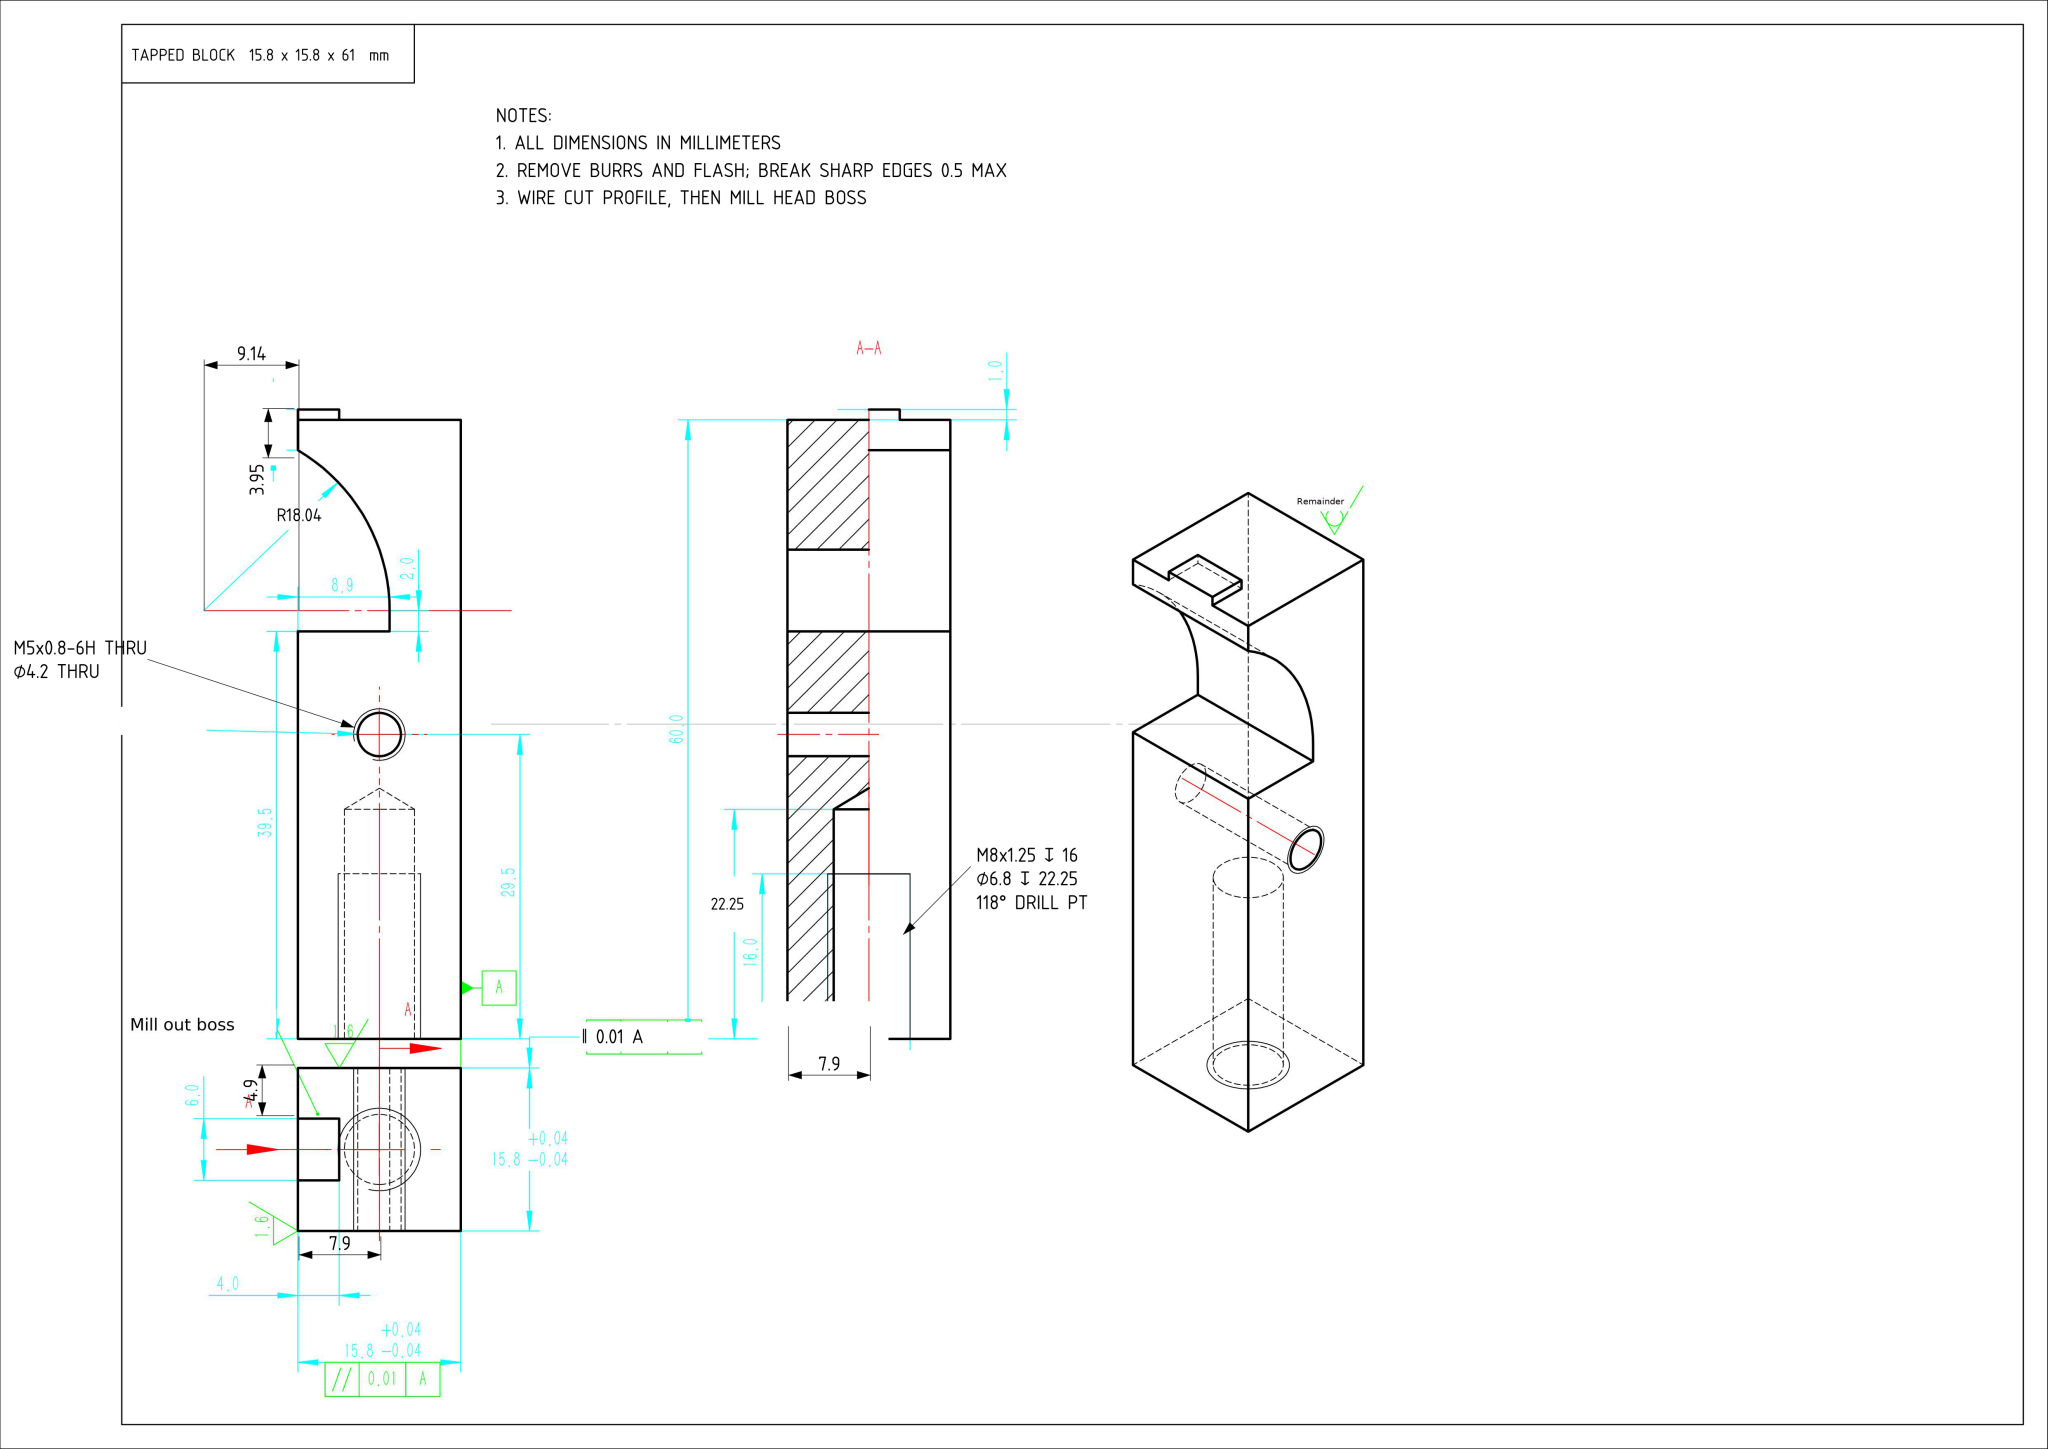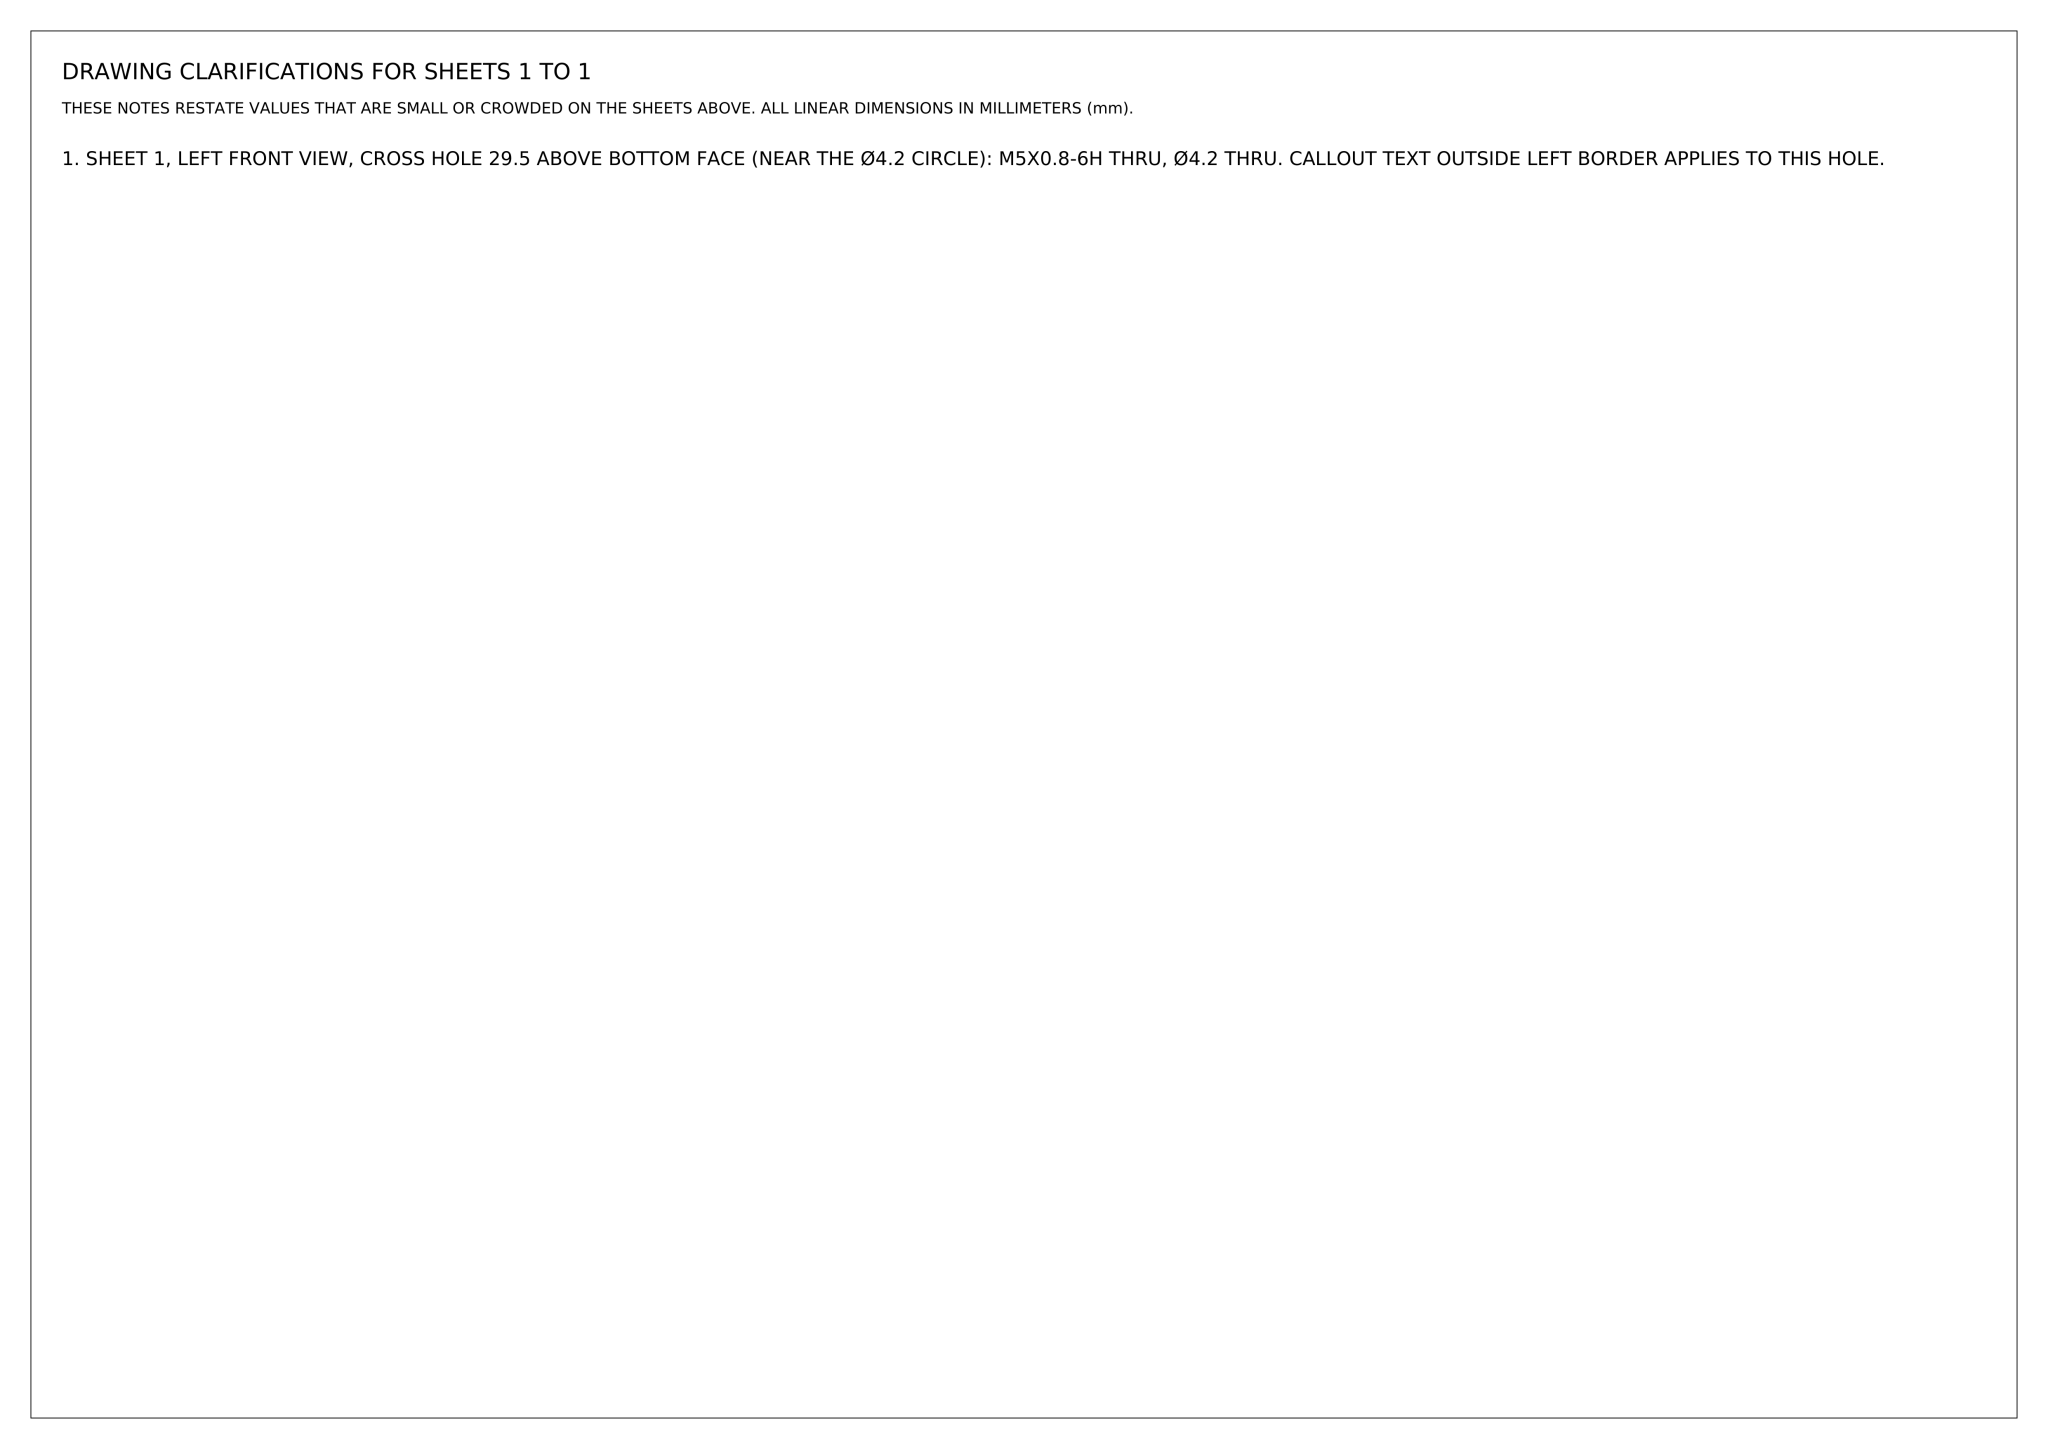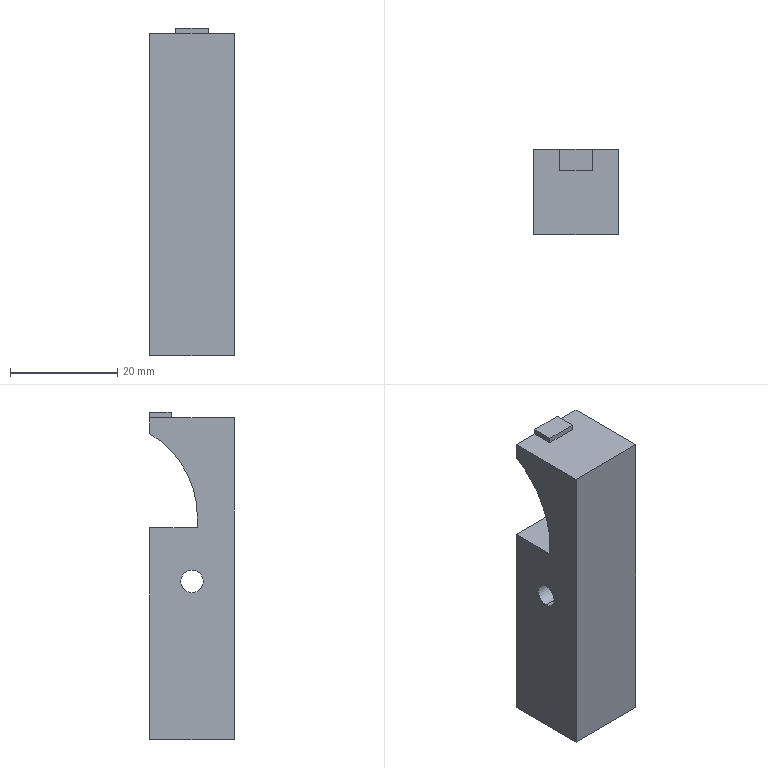Part | NX | mm | 1 solid | 20 faces | box 15.8 x 15.8 x 61 mm | volume 12120 mm3 | plane 13 | cylinder 5 | cone 2 | commonest cylinder face diameters 4.2 x2 6.8 x2 36.083 x1
STEP:
#1=COLOUR_RGB('',1.,0.651,0.);
#2=FILL_AREA_STYLE_COLOUR('',#1);
#3=FILL_AREA_STYLE('',(#2));
#4=SURFACE_STYLE_FILL_AREA(#3);
#5=SURFACE_SIDE_STYLE('',(#4));
#6=SURFACE_STYLE_USAGE(.BOTH.,#5);
#7=PRESENTATION_STYLE_ASSIGNMENT((#6));
#8=CARTESIAN_POINT('',(0.01211,-22.1,27.4));
#9=VERTEX_POINT('',#8);
#10=CARTESIAN_POINT('',(0.01211,-22.1,31.6));
#11=VERTEX_POINT('',#10);
#12=CARTESIAN_POINT('',(0.01211,-22.1,29.5));
#13=DIRECTION('',(-1.,-0.,0.));
#14=DIRECTION('',(0.,-1.,0.));
#15=AXIS2_PLACEMENT_3D('',#12,#13,#14);
#16=CIRCLE('',#15,2.1);
#17=EDGE_CURVE('',#9,#11,#16,.T.);
#18=ORIENTED_EDGE('',*,*,#17,.F.);
#19=CARTESIAN_POINT('',(-15.788,-22.1,27.4));
#20=VERTEX_POINT('',#19);
#21=CARTESIAN_POINT('',(-15.788,-22.1,27.4));
#22=DIRECTION('',(-1.,0.,0.));
#23=VECTOR('',#22,1000.);
#24=LINE('',#21,#23);
#25=EDGE_CURVE('',#9,#20,#24,.T.);
#26=ORIENTED_EDGE('',*,*,#25,.T.);
#27=CARTESIAN_POINT('',(-15.788,-22.1,31.6));
#28=VERTEX_POINT('',#27);
#29=CARTESIAN_POINT('',(-15.788,-22.1,29.5));
#30=DIRECTION('',(-1.,0.,0.));
#31=DIRECTION('',(0.,0.,1.));
#32=AXIS2_PLACEMENT_3D('',#29,#30,#31);
#33=CIRCLE('',#32,2.1);
#34=EDGE_CURVE('',#20,#28,#33,.T.);
#35=ORIENTED_EDGE('',*,*,#34,.T.);
#36=CARTESIAN_POINT('',(-15.788,-22.1,31.6));
#37=DIRECTION('',(-1.,0.,0.));
#38=VECTOR('',#37,1000.);
#39=LINE('',#36,#38);
#40=EDGE_CURVE('',#11,#28,#39,.T.);
#41=ORIENTED_EDGE('',*,*,#40,.F.);
#42=EDGE_LOOP('',(#18,#26,#35,#41));
#43=FACE_OUTER_BOUND('',#42,.T.);
#44=CARTESIAN_POINT('',(-15.788,-22.1,29.5));
#45=DIRECTION('',(-1.,0.,0.));
#46=DIRECTION('',(0.,0.,1.));
#47=AXIS2_PLACEMENT_3D('',#44,#45,#46);
#48=CYLINDRICAL_SURFACE('',#47,2.1);
#49=ADVANCED_FACE('',(#43),#48,.F.);
#50=CARTESIAN_POINT('',(-4.488,-22.1,22.25));
#51=VERTEX_POINT('',#50);
#52=CARTESIAN_POINT('',(-11.288,-22.1,22.25));
#53=VERTEX_POINT('',#52);
#54=CARTESIAN_POINT('',(-7.888,-22.1,22.25));
#55=DIRECTION('',(0.,0.,-1.));
#56=DIRECTION('',(-1.,0.,0.));
#57=AXIS2_PLACEMENT_3D('',#54,#55,#56);
#58=CIRCLE('',#57,3.4);
#59=EDGE_CURVE('',#51,#53,#58,.T.);
#60=ORIENTED_EDGE('',*,*,#59,.F.);
#61=CARTESIAN_POINT('',(-4.488,-22.1,-0.));
#62=VERTEX_POINT('',#61);
#63=CARTESIAN_POINT('',(-4.488,-22.1,0.));
#64=DIRECTION('',(0.,0.,-1.));
#65=VECTOR('',#64,1000.);
#66=LINE('',#63,#65);
#67=EDGE_CURVE('',#51,#62,#66,.T.);
#68=ORIENTED_EDGE('',*,*,#67,.T.);
#69=CARTESIAN_POINT('',(-11.288,-22.1,-0.));
#70=VERTEX_POINT('',#69);
#71=CARTESIAN_POINT('',(-7.888,-22.1,-0.));
#72=DIRECTION('',(0.,0.,-1.));
#73=DIRECTION('',(-1.,0.,0.));
#74=AXIS2_PLACEMENT_3D('',#71,#72,#73);
#75=CIRCLE('',#74,3.4);
#76=EDGE_CURVE('',#62,#70,#75,.T.);
#77=ORIENTED_EDGE('',*,*,#76,.T.);
#78=CARTESIAN_POINT('',(-11.288,-22.1,0.));
#79=DIRECTION('',(0.,0.,-1.));
#80=VECTOR('',#79,1000.);
#81=LINE('',#78,#80);
#82=EDGE_CURVE('',#53,#70,#81,.T.);
#83=ORIENTED_EDGE('',*,*,#82,.F.);
#84=EDGE_LOOP('',(#60,#68,#77,#83));
#85=FACE_OUTER_BOUND('',#84,.T.);
#86=CARTESIAN_POINT('',(-7.888,-22.1,0.));
#87=DIRECTION('',(0.,0.,-1.));
#88=DIRECTION('',(-1.,0.,0.));
#89=AXIS2_PLACEMENT_3D('',#86,#87,#88);
#90=CYLINDRICAL_SURFACE('',#89,3.4);
#91=ADVANCED_FACE('',(#85),#90,.F.);
#92=CARTESIAN_POINT('',(-7.888,-22.1,24.293));
#93=VERTEX_POINT('',#92);
#94=CARTESIAN_POINT('',(-11.288,-22.1,22.25));
#95=DIRECTION('',(-0.8572,0.,-0.515));
#96=VECTOR('',#95,1000.);
#97=LINE('',#94,#96);
#98=EDGE_CURVE('',#93,#53,#97,.T.);
#99=ORIENTED_EDGE('',*,*,#98,.F.);
#100=CARTESIAN_POINT('',(-4.488,-22.1,22.25));
#101=DIRECTION('',(0.8572,0.,-0.515));
#102=VECTOR('',#101,1000.);
#103=LINE('',#100,#102);
#104=EDGE_CURVE('',#93,#51,#103,.T.);
#105=ORIENTED_EDGE('',*,*,#104,.T.);
#106=ORIENTED_EDGE('',*,*,#59,.T.);
#107=EDGE_LOOP('',(#99,#105,#106));
#108=FACE_OUTER_BOUND('',#107,.T.);
#109=CARTESIAN_POINT('',(-7.888,-22.1,22.25));
#110=DIRECTION('',(0.,0.,-1.));
#111=DIRECTION('',(-1.,0.,0.));
#112=AXIS2_PLACEMENT_3D('',#109,#110,#111);
#113=CONICAL_SURFACE('',#112,3.4,1.03);
#114=ADVANCED_FACE('',(#108),#113,.F.);
#115=CARTESIAN_POINT('',(-10.888,-14.2,60.));
#116=VERTEX_POINT('',#115);
#117=CARTESIAN_POINT('',(-10.888,-18.2,60.));
#118=VERTEX_POINT('',#117);
#119=CARTESIAN_POINT('',(-10.888,-14.2,60.));
#120=DIRECTION('',(0.,-1.,0.));
#121=VECTOR('',#120,1000.);
#122=LINE('',#119,#121);
#123=EDGE_CURVE('',#116,#118,#122,.T.);
#124=ORIENTED_EDGE('',*,*,#123,.F.);
#125=CARTESIAN_POINT('',(-15.788,-14.2,60.));
#126=VERTEX_POINT('',#125);
#127=CARTESIAN_POINT('',(0.01211,-14.2,60.));
#128=DIRECTION('',(-1.,-0.,0.));
#129=VECTOR('',#128,1000.);
#130=LINE('',#127,#129);
#131=EDGE_CURVE('',#116,#126,#130,.T.);
#132=ORIENTED_EDGE('',*,*,#131,.T.);
#133=CARTESIAN_POINT('',(-15.788,-30.,60.));
#134=VERTEX_POINT('',#133);
#135=CARTESIAN_POINT('',(-15.788,-14.2,60.));
#136=DIRECTION('',(0.,-1.,0.));
#137=VECTOR('',#136,1000.);
#138=LINE('',#135,#137);
#139=EDGE_CURVE('',#126,#134,#138,.T.);
#140=ORIENTED_EDGE('',*,*,#139,.T.);
#141=CARTESIAN_POINT('',(0.01211,-30.,60.));
#142=VERTEX_POINT('',#141);
#143=CARTESIAN_POINT('',(0.01211,-30.,60.));
#144=DIRECTION('',(1.,0.,0.));
#145=VECTOR('',#144,1000.);
#146=LINE('',#143,#145);
#147=EDGE_CURVE('',#134,#142,#146,.T.);
#148=ORIENTED_EDGE('',*,*,#147,.T.);
#149=CARTESIAN_POINT('',(0.01211,-14.2,60.));
#150=VERTEX_POINT('',#149);
#151=CARTESIAN_POINT('',(0.01211,-14.2,60.));
#152=DIRECTION('',(-0.,1.,0.));
#153=VECTOR('',#152,1000.);
#154=LINE('',#151,#153);
#155=EDGE_CURVE('',#142,#150,#154,.T.);
#156=ORIENTED_EDGE('',*,*,#155,.T.);
#157=CARTESIAN_POINT('',(-4.888,-14.2,60.));
#158=VERTEX_POINT('',#157);
#159=CARTESIAN_POINT('',(0.01211,-14.2,60.));
#160=DIRECTION('',(-1.,-0.,0.));
#161=VECTOR('',#160,1000.);
#162=LINE('',#159,#161);
#163=EDGE_CURVE('',#150,#158,#162,.T.);
#164=ORIENTED_EDGE('',*,*,#163,.T.);
#165=CARTESIAN_POINT('',(-4.888,-18.2,60.));
#166=VERTEX_POINT('',#165);
#167=CARTESIAN_POINT('',(-4.888,-14.2,60.));
#168=DIRECTION('',(0.,-1.,0.));
#169=VECTOR('',#168,1000.);
#170=LINE('',#167,#169);
#171=EDGE_CURVE('',#158,#166,#170,.T.);
#172=ORIENTED_EDGE('',*,*,#171,.T.);
#173=CARTESIAN_POINT('',(-10.888,-18.2,60.));
#174=DIRECTION('',(1.,0.,0.));
#175=VECTOR('',#174,1000.);
#176=LINE('',#173,#175);
#177=EDGE_CURVE('',#118,#166,#176,.T.);
#178=ORIENTED_EDGE('',*,*,#177,.F.);
#179=EDGE_LOOP('',(#124,#132,#140,#148,#156,#164,#172,#178));
#180=FACE_OUTER_BOUND('',#179,.T.);
#181=CARTESIAN_POINT('',(0.,0.,60.));
#182=DIRECTION('',(0.,0.,-1.));
#183=DIRECTION('',(-1.,0.,0.));
#184=AXIS2_PLACEMENT_3D('',#181,#182,#183);
#185=PLANE('',#184);
#186=ADVANCED_FACE('',(#180),#185,.F.);
#187=CARTESIAN_POINT('',(-15.788,-23.1,41.5));
#188=VERTEX_POINT('',#187);
#189=CARTESIAN_POINT('',(-15.788,-14.2,57.054));
#190=VERTEX_POINT('',#189);
#191=CARTESIAN_POINT('',(-15.788,-5.058,41.5));
#192=DIRECTION('',(-1.,0.,0.));
#193=DIRECTION('',(0.,0.,1.));
#194=AXIS2_PLACEMENT_3D('',#191,#192,#193);
#195=CIRCLE('',#194,18.042);
#196=EDGE_CURVE('',#188,#190,#195,.T.);
#197=ORIENTED_EDGE('',*,*,#196,.F.);
#198=CARTESIAN_POINT('',(-15.788,-23.1,39.5));
#199=VERTEX_POINT('',#198);
#200=CARTESIAN_POINT('',(-15.788,-23.1,41.5));
#201=DIRECTION('',(0.,0.,1.));
#202=VECTOR('',#201,1000.);
#203=LINE('',#200,#202);
#204=EDGE_CURVE('',#199,#188,#203,.T.);
#205=ORIENTED_EDGE('',*,*,#204,.F.);
#206=CARTESIAN_POINT('',(-15.788,-14.2,39.5));
#207=VERTEX_POINT('',#206);
#208=CARTESIAN_POINT('',(-15.788,-14.2,39.5));
#209=DIRECTION('',(0.,-1.,0.));
#210=VECTOR('',#209,1000.);
#211=LINE('',#208,#210);
#212=EDGE_CURVE('',#207,#199,#211,.T.);
#213=ORIENTED_EDGE('',*,*,#212,.F.);
#214=CARTESIAN_POINT('',(-15.788,-14.2,0.));
#215=VERTEX_POINT('',#214);
#216=CARTESIAN_POINT('',(-15.788,-14.2,60.));
#217=DIRECTION('',(0.,0.,-1.));
#218=VECTOR('',#217,1000.);
#219=LINE('',#216,#218);
#220=EDGE_CURVE('',#207,#215,#219,.T.);
#221=ORIENTED_EDGE('',*,*,#220,.T.);
#222=CARTESIAN_POINT('',(-15.788,-30.,0.));
#223=VERTEX_POINT('',#222);
#224=CARTESIAN_POINT('',(-15.788,-14.2,0.));
#225=DIRECTION('',(0.,-1.,0.));
#226=VECTOR('',#225,1000.);
#227=LINE('',#224,#226);
#228=EDGE_CURVE('',#215,#223,#227,.T.);
#229=ORIENTED_EDGE('',*,*,#228,.T.);
#230=CARTESIAN_POINT('',(-15.788,-30.,60.));
#231=DIRECTION('',(0.,0.,-1.));
#232=VECTOR('',#231,1000.);
#233=LINE('',#230,#232);
#234=EDGE_CURVE('',#134,#223,#233,.T.);
#235=ORIENTED_EDGE('',*,*,#234,.F.);
#236=ORIENTED_EDGE('',*,*,#139,.F.);
#237=CARTESIAN_POINT('',(-15.788,-14.2,60.));
#238=DIRECTION('',(0.,0.,-1.));
#239=VECTOR('',#238,1000.);
#240=LINE('',#237,#239);
#241=EDGE_CURVE('',#126,#190,#240,.T.);
#242=ORIENTED_EDGE('',*,*,#241,.T.);
#243=EDGE_LOOP('',(#197,#205,#213,#221,#229,#235,#236,#242));
#244=FACE_OUTER_BOUND('',#243,.T.);
#245=CARTESIAN_POINT('',(-15.788,-22.1,29.5));
#246=DIRECTION('',(-1.,0.,0.));
#247=DIRECTION('',(0.,0.,1.));
#248=AXIS2_PLACEMENT_3D('',#245,#246,#247);
#249=CIRCLE('',#248,2.1);
#250=EDGE_CURVE('',#28,#20,#249,.T.);
#251=ORIENTED_EDGE('',*,*,#250,.F.);
#252=ORIENTED_EDGE('',*,*,#34,.F.);
#253=EDGE_LOOP('',(#251,#252));
#254=FACE_BOUND('',#253,.T.);
#255=CARTESIAN_POINT('',(-15.788,-14.2,60.));
#256=DIRECTION('',(1.,0.,0.));
#257=DIRECTION('',(0.,0.,-1.));
#258=AXIS2_PLACEMENT_3D('',#255,#256,#257);
#259=PLANE('',#258);
#260=ADVANCED_FACE('',(#244,#254),#259,.F.);
#261=CARTESIAN_POINT('',(0.01211,-14.2,57.054));
#262=VERTEX_POINT('',#261);
#263=CARTESIAN_POINT('',(0.01211,-14.2,60.));
#264=DIRECTION('',(0.,0.,-1.));
#265=VECTOR('',#264,1000.);
#266=LINE('',#263,#265);
#267=EDGE_CURVE('',#150,#262,#266,.T.);
#268=ORIENTED_EDGE('',*,*,#267,.T.);
#269=CARTESIAN_POINT('',(0.01311,-14.2,57.054));
#270=DIRECTION('',(1.,0.,0.));
#271=VECTOR('',#270,1000.);
#272=LINE('',#269,#271);
#273=EDGE_CURVE('',#190,#262,#272,.T.);
#274=ORIENTED_EDGE('',*,*,#273,.F.);
#275=ORIENTED_EDGE('',*,*,#241,.F.);
#276=ORIENTED_EDGE('',*,*,#131,.F.);
#277=CARTESIAN_POINT('',(-10.888,-14.2,61.));
#278=VERTEX_POINT('',#277);
#279=CARTESIAN_POINT('',(-10.888,-14.2,61.));
#280=DIRECTION('',(0.,0.,-1.));
#281=VECTOR('',#280,1000.);
#282=LINE('',#279,#281);
#283=EDGE_CURVE('',#278,#116,#282,.T.);
#284=ORIENTED_EDGE('',*,*,#283,.F.);
#285=CARTESIAN_POINT('',(-4.888,-14.2,61.));
#286=VERTEX_POINT('',#285);
#287=CARTESIAN_POINT('',(-10.888,-14.2,61.));
#288=DIRECTION('',(1.,0.,0.));
#289=VECTOR('',#288,1000.);
#290=LINE('',#287,#289);
#291=EDGE_CURVE('',#278,#286,#290,.T.);
#292=ORIENTED_EDGE('',*,*,#291,.T.);
#293=CARTESIAN_POINT('',(-4.888,-14.2,61.));
#294=DIRECTION('',(0.,0.,-1.));
#295=VECTOR('',#294,1000.);
#296=LINE('',#293,#295);
#297=EDGE_CURVE('',#286,#158,#296,.T.);
#298=ORIENTED_EDGE('',*,*,#297,.T.);
#299=ORIENTED_EDGE('',*,*,#163,.F.);
#300=EDGE_LOOP('',(#268,#274,#275,#276,#284,#292,#298,#299));
#301=FACE_OUTER_BOUND('',#300,.T.);
#302=CARTESIAN_POINT('',(0.01211,-14.2,60.));
#303=DIRECTION('',(0.,-1.,0.));
#304=DIRECTION('',(1.,0.,0.));
#305=AXIS2_PLACEMENT_3D('',#302,#303,#304);
#306=PLANE('',#305);
#307=ADVANCED_FACE('',(#301),#306,.F.);
#308=CARTESIAN_POINT('',(0.01211,-22.1,29.5));
#309=DIRECTION('',(-1.,-0.,0.));
#310=DIRECTION('',(0.,-1.,0.));
#311=AXIS2_PLACEMENT_3D('',#308,#309,#310);
#312=CIRCLE('',#311,2.1);
#313=EDGE_CURVE('',#11,#9,#312,.T.);
#314=ORIENTED_EDGE('',*,*,#313,.T.);
#315=ORIENTED_EDGE('',*,*,#17,.T.);
#316=EDGE_LOOP('',(#314,#315));
#317=FACE_BOUND('',#316,.T.);
#318=CARTESIAN_POINT('',(0.01211,-14.2,39.5));
#319=VERTEX_POINT('',#318);
#320=CARTESIAN_POINT('',(0.01211,-23.1,39.5));
#321=VERTEX_POINT('',#320);
#322=CARTESIAN_POINT('',(0.01211,-14.2,39.5));
#323=DIRECTION('',(0.,-1.,0.));
#324=VECTOR('',#323,1000.);
#325=LINE('',#322,#324);
#326=EDGE_CURVE('',#319,#321,#325,.T.);
#327=ORIENTED_EDGE('',*,*,#326,.T.);
#328=CARTESIAN_POINT('',(0.01211,-23.1,41.5));
#329=VERTEX_POINT('',#328);
#330=CARTESIAN_POINT('',(0.01211,-23.1,60.));
#331=DIRECTION('',(0.,0.,1.));
#332=VECTOR('',#331,1000.);
#333=LINE('',#330,#332);
#334=EDGE_CURVE('',#321,#329,#333,.T.);
#335=ORIENTED_EDGE('',*,*,#334,.T.);
#336=CARTESIAN_POINT('',(0.01211,-5.058,41.5));
#337=DIRECTION('',(1.,0.,0.));
#338=DIRECTION('',(0.,-1.,0.));
#339=AXIS2_PLACEMENT_3D('',#336,#337,#338);
#340=CIRCLE('',#339,18.042);
#341=EDGE_CURVE('',#262,#329,#340,.T.);
#342=ORIENTED_EDGE('',*,*,#341,.F.);
#343=ORIENTED_EDGE('',*,*,#267,.F.);
#344=ORIENTED_EDGE('',*,*,#155,.F.);
#345=CARTESIAN_POINT('',(0.01211,-30.,0.));
#346=VERTEX_POINT('',#345);
#347=CARTESIAN_POINT('',(0.01211,-30.,60.));
#348=DIRECTION('',(0.,0.,-1.));
#349=VECTOR('',#348,1000.);
#350=LINE('',#347,#349);
#351=EDGE_CURVE('',#142,#346,#350,.T.);
#352=ORIENTED_EDGE('',*,*,#351,.T.);
#353=CARTESIAN_POINT('',(0.01211,-14.2,0.));
#354=VERTEX_POINT('',#353);
#355=CARTESIAN_POINT('',(0.01211,-14.2,0.));
#356=DIRECTION('',(-0.,1.,0.));
#357=VECTOR('',#356,1000.);
#358=LINE('',#355,#357);
#359=EDGE_CURVE('',#346,#354,#358,.T.);
#360=ORIENTED_EDGE('',*,*,#359,.T.);
#361=CARTESIAN_POINT('',(0.01211,-14.2,60.));
#362=DIRECTION('',(0.,0.,-1.));
#363=VECTOR('',#362,1000.);
#364=LINE('',#361,#363);
#365=EDGE_CURVE('',#319,#354,#364,.T.);
#366=ORIENTED_EDGE('',*,*,#365,.F.);
#367=EDGE_LOOP('',(#327,#335,#342,#343,#344,#352,#360,#366));
#368=FACE_OUTER_BOUND('',#367,.T.);
#369=CARTESIAN_POINT('',(0.01211,-14.2,60.));
#370=DIRECTION('',(-1.,-0.,0.));
#371=DIRECTION('',(0.,-1.,0.));
#372=AXIS2_PLACEMENT_3D('',#369,#370,#371);
#373=PLANE('',#372);
#374=ADVANCED_FACE('',(#317,#368),#373,.F.);
#375=ORIENTED_EDGE('',*,*,#220,.F.);
#376=CARTESIAN_POINT('',(6.212,-14.2,39.5));
#377=DIRECTION('',(-1.,0.,0.));
#378=VECTOR('',#377,1000.);
#379=LINE('',#376,#378);
#380=EDGE_CURVE('',#319,#207,#379,.T.);
#381=ORIENTED_EDGE('',*,*,#380,.F.);
#382=ORIENTED_EDGE('',*,*,#365,.T.);
#383=CARTESIAN_POINT('',(0.01211,-14.2,0.));
#384=DIRECTION('',(-1.,-0.,0.));
#385=VECTOR('',#384,1000.);
#386=LINE('',#383,#385);
#387=EDGE_CURVE('',#354,#215,#386,.T.);
#388=ORIENTED_EDGE('',*,*,#387,.T.);
#389=EDGE_LOOP('',(#375,#381,#382,#388));
#390=FACE_OUTER_BOUND('',#389,.T.);
#391=CARTESIAN_POINT('',(0.01211,-14.2,60.));
#392=DIRECTION('',(0.,-1.,0.));
#393=DIRECTION('',(1.,0.,0.));
#394=AXIS2_PLACEMENT_3D('',#391,#392,#393);
#395=PLANE('',#394);
#396=ADVANCED_FACE('',(#390),#395,.F.);
#397=CARTESIAN_POINT('',(0.01211,-30.,0.));
#398=DIRECTION('',(1.,0.,0.));
#399=VECTOR('',#398,1000.);
#400=LINE('',#397,#399);
#401=EDGE_CURVE('',#223,#346,#400,.T.);
#402=ORIENTED_EDGE('',*,*,#401,.T.);
#403=ORIENTED_EDGE('',*,*,#351,.F.);
#404=ORIENTED_EDGE('',*,*,#147,.F.);
#405=ORIENTED_EDGE('',*,*,#234,.T.);
#406=EDGE_LOOP('',(#402,#403,#404,#405));
#407=FACE_OUTER_BOUND('',#406,.T.);
#408=CARTESIAN_POINT('',(0.01211,-30.,60.));
#409=DIRECTION('',(-0.,1.,0.));
#410=DIRECTION('',(-1.,-0.,0.));
#411=AXIS2_PLACEMENT_3D('',#408,#409,#410);
#412=PLANE('',#411);
#413=ADVANCED_FACE('',(#407),#412,.F.);
#414=CARTESIAN_POINT('',(-7.888,-22.1,-0.));
#415=DIRECTION('',(0.,0.,-1.));
#416=DIRECTION('',(-1.,0.,0.));
#417=AXIS2_PLACEMENT_3D('',#414,#415,#416);
#418=CIRCLE('',#417,3.4);
#419=EDGE_CURVE('',#70,#62,#418,.T.);
#420=ORIENTED_EDGE('',*,*,#419,.F.);
#421=ORIENTED_EDGE('',*,*,#76,.F.);
#422=EDGE_LOOP('',(#420,#421));
#423=FACE_BOUND('',#422,.T.);
#424=ORIENTED_EDGE('',*,*,#359,.F.);
#425=ORIENTED_EDGE('',*,*,#401,.F.);
#426=ORIENTED_EDGE('',*,*,#228,.F.);
#427=ORIENTED_EDGE('',*,*,#387,.F.);
#428=EDGE_LOOP('',(#424,#425,#426,#427));
#429=FACE_OUTER_BOUND('',#428,.T.);
#430=CARTESIAN_POINT('',(0.,0.,0.));
#431=DIRECTION('',(0.,0.,-1.));
#432=DIRECTION('',(-1.,0.,0.));
#433=AXIS2_PLACEMENT_3D('',#430,#431,#432);
#434=PLANE('',#433);
#435=ADVANCED_FACE('',(#423,#429),#434,.T.);
#436=ORIENTED_EDGE('',*,*,#104,.F.);
#437=ORIENTED_EDGE('',*,*,#98,.T.);
#438=CARTESIAN_POINT('',(-7.888,-22.1,22.25));
#439=DIRECTION('',(0.,0.,-1.));
#440=DIRECTION('',(-1.,0.,0.));
#441=AXIS2_PLACEMENT_3D('',#438,#439,#440);
#442=CIRCLE('',#441,3.4);
#443=EDGE_CURVE('',#53,#51,#442,.T.);
#444=ORIENTED_EDGE('',*,*,#443,.T.);
#445=EDGE_LOOP('',(#436,#437,#444));
#446=FACE_OUTER_BOUND('',#445,.T.);
#447=CARTESIAN_POINT('',(-7.888,-22.1,22.25));
#448=DIRECTION('',(0.,0.,-1.));
#449=DIRECTION('',(-1.,0.,0.));
#450=AXIS2_PLACEMENT_3D('',#447,#448,#449);
#451=CONICAL_SURFACE('',#450,3.4,1.03);
#452=ADVANCED_FACE('',(#446),#451,.F.);
#453=ORIENTED_EDGE('',*,*,#67,.F.);
#454=ORIENTED_EDGE('',*,*,#443,.F.);
#455=ORIENTED_EDGE('',*,*,#82,.T.);
#456=ORIENTED_EDGE('',*,*,#419,.T.);
#457=EDGE_LOOP('',(#453,#454,#455,#456));
#458=FACE_OUTER_BOUND('',#457,.T.);
#459=CARTESIAN_POINT('',(-7.888,-22.1,0.));
#460=DIRECTION('',(0.,0.,-1.));
#461=DIRECTION('',(-1.,0.,0.));
#462=AXIS2_PLACEMENT_3D('',#459,#460,#461);
#463=CYLINDRICAL_SURFACE('',#462,3.4);
#464=ADVANCED_FACE('',(#458),#463,.F.);
#465=ORIENTED_EDGE('',*,*,#341,.T.);
#466=CARTESIAN_POINT('',(0.01311,-23.1,41.5));
#467=DIRECTION('',(-1.,0.,0.));
#468=VECTOR('',#467,1000.);
#469=LINE('',#466,#468);
#470=EDGE_CURVE('',#329,#188,#469,.T.);
#471=ORIENTED_EDGE('',*,*,#470,.T.);
#472=ORIENTED_EDGE('',*,*,#196,.T.);
#473=ORIENTED_EDGE('',*,*,#273,.T.);
#474=EDGE_LOOP('',(#465,#471,#472,#473));
#475=FACE_OUTER_BOUND('',#474,.T.);
#476=CARTESIAN_POINT('',(0.01311,-5.058,41.5));
#477=DIRECTION('',(-1.,0.,0.));
#478=DIRECTION('',(0.,0.,1.));
#479=AXIS2_PLACEMENT_3D('',#476,#477,#478);
#480=CYLINDRICAL_SURFACE('',#479,18.042);
#481=ADVANCED_FACE('',(#475),#480,.F.);
#482=ORIENTED_EDGE('',*,*,#25,.F.);
#483=ORIENTED_EDGE('',*,*,#313,.F.);
#484=ORIENTED_EDGE('',*,*,#40,.T.);
#485=ORIENTED_EDGE('',*,*,#250,.T.);
#486=EDGE_LOOP('',(#482,#483,#484,#485));
#487=FACE_OUTER_BOUND('',#486,.T.);
#488=CARTESIAN_POINT('',(-15.788,-22.1,29.5));
#489=DIRECTION('',(-1.,0.,0.));
#490=DIRECTION('',(0.,0.,1.));
#491=AXIS2_PLACEMENT_3D('',#488,#489,#490);
#492=CYLINDRICAL_SURFACE('',#491,2.1);
#493=ADVANCED_FACE('',(#487),#492,.F.);
#494=ORIENTED_EDGE('',*,*,#123,.T.);
#495=CARTESIAN_POINT('',(-10.888,-18.2,61.));
#496=VERTEX_POINT('',#495);
#497=CARTESIAN_POINT('',(-10.888,-18.2,61.));
#498=DIRECTION('',(0.,0.,-1.));
#499=VECTOR('',#498,1000.);
#500=LINE('',#497,#499);
#501=EDGE_CURVE('',#496,#118,#500,.T.);
#502=ORIENTED_EDGE('',*,*,#501,.F.);
#503=CARTESIAN_POINT('',(-10.888,-14.2,61.));
#504=DIRECTION('',(0.,-1.,0.));
#505=VECTOR('',#504,1000.);
#506=LINE('',#503,#505);
#507=EDGE_CURVE('',#278,#496,#506,.T.);
#508=ORIENTED_EDGE('',*,*,#507,.F.);
#509=ORIENTED_EDGE('',*,*,#283,.T.);
#510=EDGE_LOOP('',(#494,#502,#508,#509));
#511=FACE_OUTER_BOUND('',#510,.T.);
#512=CARTESIAN_POINT('',(-10.888,-14.2,61.));
#513=DIRECTION('',(1.,0.,0.));
#514=DIRECTION('',(0.,0.,-1.));
#515=AXIS2_PLACEMENT_3D('',#512,#513,#514);
#516=PLANE('',#515);
#517=ADVANCED_FACE('',(#511),#516,.F.);
#518=ORIENTED_EDGE('',*,*,#177,.T.);
#519=CARTESIAN_POINT('',(-4.888,-18.2,61.));
#520=VERTEX_POINT('',#519);
#521=CARTESIAN_POINT('',(-4.888,-18.2,61.));
#522=DIRECTION('',(0.,0.,-1.));
#523=VECTOR('',#522,1000.);
#524=LINE('',#521,#523);
#525=EDGE_CURVE('',#520,#166,#524,.T.);
#526=ORIENTED_EDGE('',*,*,#525,.F.);
#527=CARTESIAN_POINT('',(-10.888,-18.2,61.));
#528=DIRECTION('',(1.,0.,0.));
#529=VECTOR('',#528,1000.);
#530=LINE('',#527,#529);
#531=EDGE_CURVE('',#496,#520,#530,.T.);
#532=ORIENTED_EDGE('',*,*,#531,.F.);
#533=ORIENTED_EDGE('',*,*,#501,.T.);
#534=EDGE_LOOP('',(#518,#526,#532,#533));
#535=FACE_OUTER_BOUND('',#534,.T.);
#536=CARTESIAN_POINT('',(-10.888,-18.2,61.));
#537=DIRECTION('',(0.,1.,0.));
#538=DIRECTION('',(0.,0.,1.));
#539=AXIS2_PLACEMENT_3D('',#536,#537,#538);
#540=PLANE('',#539);
#541=ADVANCED_FACE('',(#535),#540,.F.);
#542=ORIENTED_EDGE('',*,*,#171,.F.);
#543=ORIENTED_EDGE('',*,*,#297,.F.);
#544=CARTESIAN_POINT('',(-4.888,-14.2,61.));
#545=DIRECTION('',(0.,-1.,0.));
#546=VECTOR('',#545,1000.);
#547=LINE('',#544,#546);
#548=EDGE_CURVE('',#286,#520,#547,.T.);
#549=ORIENTED_EDGE('',*,*,#548,.T.);
#550=ORIENTED_EDGE('',*,*,#525,.T.);
#551=EDGE_LOOP('',(#542,#543,#549,#550));
#552=FACE_OUTER_BOUND('',#551,.T.);
#553=CARTESIAN_POINT('',(-4.888,-14.2,61.));
#554=DIRECTION('',(1.,0.,0.));
#555=DIRECTION('',(-0.,1.,0.));
#556=AXIS2_PLACEMENT_3D('',#553,#554,#555);
#557=PLANE('',#556);
#558=ADVANCED_FACE('',(#552),#557,.T.);
#559=ORIENTED_EDGE('',*,*,#507,.T.);
#560=ORIENTED_EDGE('',*,*,#531,.T.);
#561=ORIENTED_EDGE('',*,*,#548,.F.);
#562=ORIENTED_EDGE('',*,*,#291,.F.);
#563=EDGE_LOOP('',(#559,#560,#561,#562));
#564=FACE_OUTER_BOUND('',#563,.T.);
#565=CARTESIAN_POINT('',(0.,0.,61.));
#566=DIRECTION('',(0.,0.,1.));
#567=DIRECTION('',(1.,0.,0.));
#568=AXIS2_PLACEMENT_3D('',#565,#566,#567);
#569=PLANE('',#568);
#570=ADVANCED_FACE('',(#564),#569,.T.);
#571=ORIENTED_EDGE('',*,*,#380,.T.);
#572=ORIENTED_EDGE('',*,*,#212,.T.);
#573=CARTESIAN_POINT('',(6.212,-23.1,39.5));
#574=DIRECTION('',(-1.,0.,0.));
#575=VECTOR('',#574,1000.);
#576=LINE('',#573,#575);
#577=EDGE_CURVE('',#321,#199,#576,.T.);
#578=ORIENTED_EDGE('',*,*,#577,.F.);
#579=ORIENTED_EDGE('',*,*,#326,.F.);
#580=EDGE_LOOP('',(#571,#572,#578,#579));
#581=FACE_OUTER_BOUND('',#580,.T.);
#582=CARTESIAN_POINT('',(6.212,-14.2,39.5));
#583=DIRECTION('',(0.,0.,-1.));
#584=DIRECTION('',(-1.,0.,0.));
#585=AXIS2_PLACEMENT_3D('',#582,#583,#584);
#586=PLANE('',#585);
#587=ADVANCED_FACE('',(#581),#586,.F.);
#588=ORIENTED_EDGE('',*,*,#577,.T.);
#589=ORIENTED_EDGE('',*,*,#204,.T.);
#590=ORIENTED_EDGE('',*,*,#470,.F.);
#591=ORIENTED_EDGE('',*,*,#334,.F.);
#592=EDGE_LOOP('',(#588,#589,#590,#591));
#593=FACE_OUTER_BOUND('',#592,.T.);
#594=CARTESIAN_POINT('',(6.212,-23.1,41.5));
#595=DIRECTION('',(0.,-1.,0.));
#596=DIRECTION('',(0.,0.,-1.));
#597=AXIS2_PLACEMENT_3D('',#594,#595,#596);
#598=PLANE('',#597);
#599=ADVANCED_FACE('',(#593),#598,.F.);
#600=CLOSED_SHELL('',(#49,#91,#114,#186,#260,#307,#374,#396,#413,#435,#452,#464,#481,#493,#517,#541,#558,#570,#587,#599));
#601=MANIFOLD_SOLID_BREP('',#600);
#602=CARTESIAN_POINT('',(0.,0.,0.));
#603=DIRECTION('',(0.,0.,1.));
#604=DIRECTION('',(1.,0.,0.));
#605=AXIS2_PLACEMENT_3D('',#602,#603,#604);
#606=(LENGTH_UNIT()NAMED_UNIT(*)SI_UNIT(.MILLI.,.METRE.));
#607=UNCERTAINTY_MEASURE_WITH_UNIT(LENGTH_MEASURE(0.00001),#606,'','');
#608=(NAMED_UNIT(*)PLANE_ANGLE_UNIT()SI_UNIT($,.RADIAN.));
#609=(NAMED_UNIT(*)SI_UNIT($,.STERADIAN.)SOLID_ANGLE_UNIT());
#610=(GEOMETRIC_REPRESENTATION_CONTEXT(3)GLOBAL_UNCERTAINTY_ASSIGNED_CONTEXT((#607))GLOBAL_UNIT_ASSIGNED_CONTEXT((#606,#608,#609))REPRESENTATION_CONTEXT('',''));
#611=ADVANCED_BREP_SHAPE_REPRESENTATION('',(#601,#605),#610);
#612=STYLED_ITEM('',(#7),#611);
#613=PRESENTATION_LAYER_ASSIGNMENT('','',(#612));
#614=COLOUR_RGB('',0.6157,0.6431,0.6745);
#615=FILL_AREA_STYLE_COLOUR('',#614);
#616=FILL_AREA_STYLE('',(#615));
#617=SURFACE_STYLE_FILL_AREA(#616);
#618=SURFACE_SIDE_STYLE('',(#617));
#619=SURFACE_STYLE_USAGE(.BOTH.,#618);
#620=PRESENTATION_STYLE_ASSIGNMENT((#619));
#621=STYLED_ITEM('',(#620),#493);
#622=(LENGTH_UNIT()NAMED_UNIT(*)SI_UNIT(.MILLI.,.METRE.));
#623=UNCERTAINTY_MEASURE_WITH_UNIT(LENGTH_MEASURE(0.00001),#622,'','');
#624=(NAMED_UNIT(*)PLANE_ANGLE_UNIT()SI_UNIT($,.RADIAN.));
#625=(NAMED_UNIT(*)SI_UNIT($,.STERADIAN.)SOLID_ANGLE_UNIT());
#626=(GEOMETRIC_REPRESENTATION_CONTEXT(3)GLOBAL_UNCERTAINTY_ASSIGNED_CONTEXT((#623))GLOBAL_UNIT_ASSIGNED_CONTEXT((#622,#624,#625))REPRESENTATION_CONTEXT('',''));
#627=MECHANICAL_DESIGN_GEOMETRIC_PRESENTATION_REPRESENTATION('',(#621),#626);
#628=COLOUR_RGB('',1.,0.651,0.);
#629=FILL_AREA_STYLE_COLOUR('',#628);
#630=FILL_AREA_STYLE('',(#629));
#631=SURFACE_STYLE_FILL_AREA(#630);
#632=SURFACE_SIDE_STYLE('',(#631));
#633=SURFACE_STYLE_USAGE(.BOTH.,#632);
#634=PRESENTATION_STYLE_ASSIGNMENT((#633));
#635=STYLED_ITEM('',(#634),#601);
#636=(LENGTH_UNIT()NAMED_UNIT(*)SI_UNIT(.MILLI.,.METRE.));
#637=UNCERTAINTY_MEASURE_WITH_UNIT(LENGTH_MEASURE(0.00001),#636,'','');
#638=(NAMED_UNIT(*)PLANE_ANGLE_UNIT()SI_UNIT($,.RADIAN.));
#639=(NAMED_UNIT(*)SI_UNIT($,.STERADIAN.)SOLID_ANGLE_UNIT());
#640=(GEOMETRIC_REPRESENTATION_CONTEXT(3)GLOBAL_UNCERTAINTY_ASSIGNED_CONTEXT((#637))GLOBAL_UNIT_ASSIGNED_CONTEXT((#636,#638,#639))REPRESENTATION_CONTEXT('',''));
#641=MECHANICAL_DESIGN_GEOMETRIC_PRESENTATION_REPRESENTATION('',(#635),#640);
#642=PRESENTATION_LAYER_ASSIGNMENT('','',(#635));
#643=COLOUR_RGB('',0.6157,0.6431,0.6745);
#644=FILL_AREA_STYLE_COLOUR('',#643);
#645=FILL_AREA_STYLE('',(#644));
#646=SURFACE_STYLE_FILL_AREA(#645);
#647=SURFACE_SIDE_STYLE('',(#646));
#648=SURFACE_STYLE_USAGE(.BOTH.,#647);
#649=PRESENTATION_STYLE_ASSIGNMENT((#648));
#650=STYLED_ITEM('',(#649),#49);
#651=PRESENTATION_LAYER_ASSIGNMENT('','',(#650));
#652=PRESENTATION_LAYER_ASSIGNMENT('','',(#621));
#653=COLOUR_RGB('',0.6157,0.6431,0.6745);
#654=FILL_AREA_STYLE_COLOUR('',#653);
#655=FILL_AREA_STYLE('',(#654));
#656=SURFACE_STYLE_FILL_AREA(#655);
#657=SURFACE_SIDE_STYLE('',(#656));
#658=SURFACE_STYLE_USAGE(.BOTH.,#657);
#659=PRESENTATION_STYLE_ASSIGNMENT((#658));
#660=STYLED_ITEM('',(#659),#91);
#661=(LENGTH_UNIT()NAMED_UNIT(*)SI_UNIT(.MILLI.,.METRE.));
#662=UNCERTAINTY_MEASURE_WITH_UNIT(LENGTH_MEASURE(0.00001),#661,'','');
#663=(NAMED_UNIT(*)PLANE_ANGLE_UNIT()SI_UNIT($,.RADIAN.));
#664=(NAMED_UNIT(*)SI_UNIT($,.STERADIAN.)SOLID_ANGLE_UNIT());
#665=(GEOMETRIC_REPRESENTATION_CONTEXT(3)GLOBAL_UNCERTAINTY_ASSIGNED_CONTEXT((#662))GLOBAL_UNIT_ASSIGNED_CONTEXT((#661,#663,#664))REPRESENTATION_CONTEXT('',''));
#666=MECHANICAL_DESIGN_GEOMETRIC_PRESENTATION_REPRESENTATION('',(#660),#665);
#667=PRESENTATION_LAYER_ASSIGNMENT('','',(#660));
#668=COLOUR_RGB('',0.6157,0.6431,0.6745);
#669=FILL_AREA_STYLE_COLOUR('',#668);
#670=FILL_AREA_STYLE('',(#669));
#671=SURFACE_STYLE_FILL_AREA(#670);
#672=SURFACE_SIDE_STYLE('',(#671));
#673=SURFACE_STYLE_USAGE(.BOTH.,#672);
#674=PRESENTATION_STYLE_ASSIGNMENT((#673));
#675=STYLED_ITEM('',(#674),#464);
#676=(LENGTH_UNIT()NAMED_UNIT(*)SI_UNIT(.MILLI.,.METRE.));
#677=UNCERTAINTY_MEASURE_WITH_UNIT(LENGTH_MEASURE(0.00001),#676,'','');
#678=(NAMED_UNIT(*)PLANE_ANGLE_UNIT()SI_UNIT($,.RADIAN.));
#679=(NAMED_UNIT(*)SI_UNIT($,.STERADIAN.)SOLID_ANGLE_UNIT());
#680=(GEOMETRIC_REPRESENTATION_CONTEXT(3)GLOBAL_UNCERTAINTY_ASSIGNED_CONTEXT((#677))GLOBAL_UNIT_ASSIGNED_CONTEXT((#676,#678,#679))REPRESENTATION_CONTEXT('',''));
#681=MECHANICAL_DESIGN_GEOMETRIC_PRESENTATION_REPRESENTATION('',(#675),#680);
#682=PRESENTATION_LAYER_ASSIGNMENT('','',(#675));
#683=(LENGTH_UNIT()NAMED_UNIT(*)SI_UNIT(.MILLI.,.METRE.));
#684=UNCERTAINTY_MEASURE_WITH_UNIT(LENGTH_MEASURE(0.00001),#683,'','');
#685=(NAMED_UNIT(*)PLANE_ANGLE_UNIT()SI_UNIT($,.RADIAN.));
#686=(NAMED_UNIT(*)SI_UNIT($,.STERADIAN.)SOLID_ANGLE_UNIT());
#687=(GEOMETRIC_REPRESENTATION_CONTEXT(3)GLOBAL_UNCERTAINTY_ASSIGNED_CONTEXT((#684))GLOBAL_UNIT_ASSIGNED_CONTEXT((#683,#685,#686))REPRESENTATION_CONTEXT('',''));
#688=MECHANICAL_DESIGN_GEOMETRIC_PRESENTATION_REPRESENTATION('',(#650),#687);
#689=(LENGTH_UNIT()NAMED_UNIT(*)SI_UNIT(.MILLI.,.METRE.));
#690=UNCERTAINTY_MEASURE_WITH_UNIT(LENGTH_MEASURE(0.00001),#689,'','');
#691=(NAMED_UNIT(*)PLANE_ANGLE_UNIT()SI_UNIT($,.RADIAN.));
#692=(NAMED_UNIT(*)SI_UNIT($,.STERADIAN.)SOLID_ANGLE_UNIT());
#693=(GEOMETRIC_REPRESENTATION_CONTEXT(3)GLOBAL_UNCERTAINTY_ASSIGNED_CONTEXT((#690))GLOBAL_UNIT_ASSIGNED_CONTEXT((#689,#691,#692))REPRESENTATION_CONTEXT('',''));
#694=MECHANICAL_DESIGN_GEOMETRIC_PRESENTATION_REPRESENTATION('',(#612),#693);